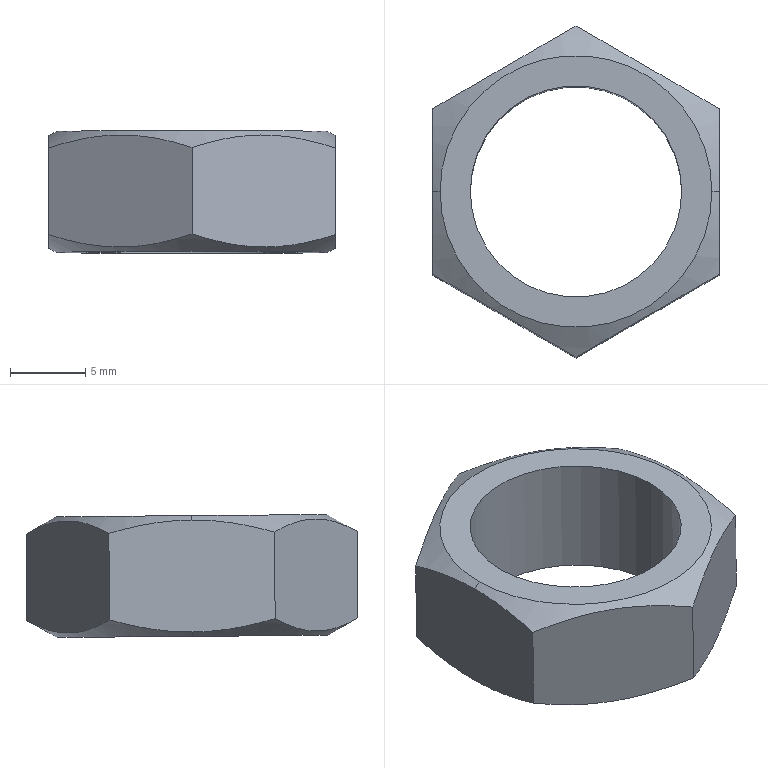Component | SolidWorks | CG1UN40-50Nut-1 | 1 solid | 14 faces | box 19 x 21.98 x 8.14 mm | volume 1229 mm3 | plane 8 | cone 4 | cylinder 2 | commonest cylinder face diameters 14 x2
STEP:
#1=CARTESIAN_POINT('',(7.598,4.142,0.1182));
#2=VERTEX_POINT('',#1);
#3=CARTESIAN_POINT('',(8.15,4.142,0.1182));
#4=VERTEX_POINT('',#3);
#5=CARTESIAN_POINT('',(7.874,4.142,0.1182));
#6=DIRECTION('',(-0.,0.008055,1.));
#7=DIRECTION('',(-1.,0.,-0.));
#8=AXIS2_PLACEMENT_3D('',#5,#6,#7);
#9=CIRCLE('',#8,0.2756);
#10=EDGE_CURVE('',#2,#4,#9,.T.);
#11=ORIENTED_EDGE('',*,*,#10,.F.);
#12=CARTESIAN_POINT('',(7.598,4.145,0.4332));
#13=VERTEX_POINT('',#12);
#14=CARTESIAN_POINT('',(7.598,4.144,0.2757));
#15=DIRECTION('',(-0.,0.008055,1.));
#16=VECTOR('',#15,39.37);
#17=LINE('',#14,#16);
#18=EDGE_CURVE('',#2,#13,#17,.T.);
#19=ORIENTED_EDGE('',*,*,#18,.T.);
#20=CARTESIAN_POINT('',(8.15,4.145,0.4332));
#21=VERTEX_POINT('',#20);
#22=CARTESIAN_POINT('',(7.874,4.145,0.4332));
#23=DIRECTION('',(0.,-0.008055,-1.));
#24=DIRECTION('',(1.,-0.,0.));
#25=AXIS2_PLACEMENT_3D('',#22,#23,#24);
#26=CIRCLE('',#25,0.2756);
#27=EDGE_CURVE('',#21,#13,#26,.T.);
#28=ORIENTED_EDGE('',*,*,#27,.F.);
#29=CARTESIAN_POINT('',(8.15,4.144,0.2757));
#30=DIRECTION('',(-0.,0.008055,1.));
#31=VECTOR('',#30,39.37);
#32=LINE('',#29,#31);
#33=EDGE_CURVE('',#4,#21,#32,.T.);
#34=ORIENTED_EDGE('',*,*,#33,.F.);
#35=EDGE_LOOP('',(#11,#19,#28,#34));
#36=FACE_OUTER_BOUND('',#35,.T.);
#37=CARTESIAN_POINT('',(7.874,4.144,0.2757));
#38=DIRECTION('',(-0.,0.008055,1.));
#39=DIRECTION('',(1.,0.,0.));
#40=AXIS2_PLACEMENT_3D('',#37,#38,#39);
#41=CYLINDRICAL_SURFACE('',#40,0.2756);
#42=ADVANCED_FACE('',(#36),#41,.F.);
#43=CARTESIAN_POINT('',(8.228,4.142,0.1182));
#44=VERTEX_POINT('',#43);
#45=CARTESIAN_POINT('',(7.52,4.142,0.1182));
#46=VERTEX_POINT('',#45);
#47=CARTESIAN_POINT('',(7.874,4.142,0.1182));
#48=DIRECTION('',(-0.,0.008055,1.));
#49=DIRECTION('',(1.,0.,0.));
#50=AXIS2_PLACEMENT_3D('',#47,#48,#49);
#51=CIRCLE('',#50,0.3543);
#52=EDGE_CURVE('',#44,#46,#51,.T.);
#53=ORIENTED_EDGE('',*,*,#52,.T.);
#54=CARTESIAN_POINT('',(7.5,4.142,0.1296));
#55=VERTEX_POINT('',#54);
#56=CARTESIAN_POINT('',(7.442,4.143,0.1633));
#57=DIRECTION('',(-0.866,0.004027,0.5));
#58=VECTOR('',#57,39.37);
#59=LINE('',#56,#58);
#60=EDGE_CURVE('',#46,#55,#59,.T.);
#61=ORIENTED_EDGE('',*,*,#60,.T.);
#62=CARTESIAN_POINT('',(7.5,4.359,0.1613));
#63=VERTEX_POINT('',#62);
#64=CARTESIAN_POINT('',(7.5,4.142,0.1296));
#65=CARTESIAN_POINT('',(7.5,4.161,0.1295));
#66=CARTESIAN_POINT('',(7.5,4.179,0.1301));
#67=CARTESIAN_POINT('',(7.5,4.216,0.1329));
#68=CARTESIAN_POINT('',(7.5,4.234,0.135));
#69=CARTESIAN_POINT('',(7.5,4.288,0.1433));
#70=CARTESIAN_POINT('',(7.5,4.323,0.1514));
#71=CARTESIAN_POINT('',(7.5,4.359,0.1613));
#72=B_SPLINE_CURVE_WITH_KNOTS('',3,(#64,#65,#66,#67,#68,#69,#70,#71),.UNSPECIFIED.,.F.,.F.,(4,2,2,4),(0.00555,0.006932,0.008314,0.01108),.UNSPECIFIED.);
#73=EDGE_CURVE('',#55,#63,#72,.T.);
#74=ORIENTED_EDGE('',*,*,#73,.T.);
#75=CARTESIAN_POINT('',(7.874,4.575,0.1595));
#76=VERTEX_POINT('',#75);
#77=CARTESIAN_POINT('',(7.5,4.359,0.1613));
#78=CARTESIAN_POINT('',(7.531,4.376,0.1509));
#79=CARTESIAN_POINT('',(7.561,4.394,0.1424));
#80=CARTESIAN_POINT('',(7.623,4.43,0.1305));
#81=CARTESIAN_POINT('',(7.655,4.448,0.1272));
#82=CARTESIAN_POINT('',(7.703,4.475,0.1269));
#83=CARTESIAN_POINT('',(7.719,4.484,0.1276));
#84=CARTESIAN_POINT('',(7.75,4.503,0.1305));
#85=CARTESIAN_POINT('',(7.766,4.512,0.1327));
#86=CARTESIAN_POINT('',(7.813,4.539,0.1412));
#87=CARTESIAN_POINT('',(7.843,4.557,0.1495));
#88=CARTESIAN_POINT('',(7.874,4.575,0.1595));
#89=B_SPLINE_CURVE_WITH_KNOTS('',3,(#77,#78,#79,#80,#81,#82,#83,#84,#85,#86,#87,#88),.UNSPECIFIED.,.F.,.F.,(4,2,2,2,2,4),(0.,0.00277,0.005539,0.006924,0.008309,0.01108),.UNSPECIFIED.);
#90=EDGE_CURVE('',#63,#76,#89,.T.);
#91=ORIENTED_EDGE('',*,*,#90,.T.);
#92=CARTESIAN_POINT('',(8.248,4.359,0.1613));
#93=VERTEX_POINT('',#92);
#94=CARTESIAN_POINT('',(7.874,4.575,0.1595));
#95=CARTESIAN_POINT('',(7.905,4.557,0.1495));
#96=CARTESIAN_POINT('',(7.935,4.539,0.1412));
#97=CARTESIAN_POINT('',(7.997,4.503,0.1299));
#98=CARTESIAN_POINT('',(8.029,4.485,0.1269));
#99=CARTESIAN_POINT('',(8.077,4.457,0.1271));
#100=CARTESIAN_POINT('',(8.093,4.448,0.1279));
#101=CARTESIAN_POINT('',(8.124,4.43,0.1311));
#102=CARTESIAN_POINT('',(8.14,4.421,0.1334));
#103=CARTESIAN_POINT('',(8.187,4.394,0.1424));
#104=CARTESIAN_POINT('',(8.217,4.376,0.1509));
#105=CARTESIAN_POINT('',(8.248,4.359,0.1613));
#106=B_SPLINE_CURVE_WITH_KNOTS('',3,(#94,#95,#96,#97,#98,#99,#100,#101,#102,#103,#104,#105),.UNSPECIFIED.,.F.,.F.,(4,2,2,2,2,4),(0.,0.00277,0.005539,0.006924,0.008309,0.01108),.UNSPECIFIED.);
#107=EDGE_CURVE('',#76,#93,#106,.T.);
#108=ORIENTED_EDGE('',*,*,#107,.T.);
#109=CARTESIAN_POINT('',(8.248,4.142,0.1296));
#110=VERTEX_POINT('',#109);
#111=CARTESIAN_POINT('',(8.248,4.359,0.1613));
#112=CARTESIAN_POINT('',(8.248,4.323,0.1514));
#113=CARTESIAN_POINT('',(8.248,4.288,0.1432));
#114=CARTESIAN_POINT('',(8.248,4.216,0.1322));
#115=CARTESIAN_POINT('',(8.248,4.179,0.1293));
#116=CARTESIAN_POINT('',(8.248,4.142,0.1296));
#117=B_SPLINE_CURVE_WITH_KNOTS('',3,(#111,#112,#113,#114,#115,#116),.UNSPECIFIED.,.F.,.F.,(4,2,4),(0.,0.002775,0.00555),.UNSPECIFIED.);
#118=EDGE_CURVE('',#93,#110,#117,.T.);
#119=ORIENTED_EDGE('',*,*,#118,.T.);
#120=CARTESIAN_POINT('',(8.306,4.143,0.1633));
#121=DIRECTION('',(0.866,0.004027,0.5));
#122=VECTOR('',#121,39.37);
#123=LINE('',#120,#122);
#124=EDGE_CURVE('',#44,#110,#123,.T.);
#125=ORIENTED_EDGE('',*,*,#124,.F.);
#126=EDGE_LOOP('',(#53,#61,#74,#91,#108,#119,#125));
#127=FACE_OUTER_BOUND('',#126,.T.);
#128=CARTESIAN_POINT('',(7.874,4.143,0.1633));
#129=DIRECTION('',(-0.,0.008055,1.));
#130=DIRECTION('',(1.,0.,0.));
#131=AXIS2_PLACEMENT_3D('',#128,#129,#130);
#132=CONICAL_SURFACE('',#131,0.4323,1.047);
#133=ADVANCED_FACE('',(#127),#132,.T.);
#134=CARTESIAN_POINT('',(8.228,4.145,0.4332));
#135=VERTEX_POINT('',#134);
#136=CARTESIAN_POINT('',(7.52,4.145,0.4332));
#137=VERTEX_POINT('',#136);
#138=CARTESIAN_POINT('',(7.874,4.145,0.4332));
#139=DIRECTION('',(-0.,0.008055,1.));
#140=DIRECTION('',(-1.,0.,-0.));
#141=AXIS2_PLACEMENT_3D('',#138,#139,#140);
#142=CIRCLE('',#141,0.3543);
#143=EDGE_CURVE('',#135,#137,#142,.T.);
#144=ORIENTED_EDGE('',*,*,#143,.F.);
#145=CARTESIAN_POINT('',(8.248,4.145,0.4218));
#146=VERTEX_POINT('',#145);
#147=CARTESIAN_POINT('',(8.306,4.144,0.3881));
#148=DIRECTION('',(0.866,-0.004027,-0.5));
#149=VECTOR('',#148,39.37);
#150=LINE('',#147,#149);
#151=EDGE_CURVE('',#135,#146,#150,.T.);
#152=ORIENTED_EDGE('',*,*,#151,.T.);
#153=CARTESIAN_POINT('',(8.248,4.36,0.3867));
#154=VERTEX_POINT('',#153);
#155=CARTESIAN_POINT('',(8.248,4.145,0.4218));
#156=CARTESIAN_POINT('',(8.248,4.163,0.4217));
#157=CARTESIAN_POINT('',(8.248,4.181,0.4207));
#158=CARTESIAN_POINT('',(8.248,4.218,0.4174));
#159=CARTESIAN_POINT('',(8.248,4.236,0.415));
#160=CARTESIAN_POINT('',(8.248,4.29,0.4058));
#161=CARTESIAN_POINT('',(8.248,4.325,0.3971));
#162=CARTESIAN_POINT('',(8.248,4.36,0.3867));
#163=B_SPLINE_CURVE_WITH_KNOTS('',3,(#155,#156,#157,#158,#159,#160,#161,#162),.UNSPECIFIED.,.F.,.F.,(4,2,2,4),(0.00555,0.006932,0.008314,0.01108),.UNSPECIFIED.);
#164=EDGE_CURVE('',#146,#154,#163,.T.);
#165=ORIENTED_EDGE('',*,*,#164,.T.);
#166=CARTESIAN_POINT('',(7.874,4.576,0.3849));
#167=VERTEX_POINT('',#166);
#168=CARTESIAN_POINT('',(8.248,4.36,0.3867));
#169=CARTESIAN_POINT('',(8.217,4.378,0.3967));
#170=CARTESIAN_POINT('',(8.187,4.396,0.405));
#171=CARTESIAN_POINT('',(8.125,4.432,0.4163));
#172=CARTESIAN_POINT('',(8.093,4.45,0.4193));
#173=CARTESIAN_POINT('',(8.045,4.478,0.4192));
#174=CARTESIAN_POINT('',(8.03,4.487,0.4183));
#175=CARTESIAN_POINT('',(7.998,4.505,0.4151));
#176=CARTESIAN_POINT('',(7.982,4.514,0.4128));
#177=CARTESIAN_POINT('',(7.935,4.541,0.4038));
#178=CARTESIAN_POINT('',(7.905,4.559,0.3953));
#179=CARTESIAN_POINT('',(7.874,4.576,0.3849));
#180=B_SPLINE_CURVE_WITH_KNOTS('',3,(#168,#169,#170,#171,#172,#173,#174,#175,#176,#177,#178,#179),.UNSPECIFIED.,.F.,.F.,(4,2,2,2,2,4),(0.,0.00277,0.005539,0.006924,0.008309,0.01108),.UNSPECIFIED.);
#181=EDGE_CURVE('',#154,#167,#180,.T.);
#182=ORIENTED_EDGE('',*,*,#181,.T.);
#183=CARTESIAN_POINT('',(7.5,4.36,0.3867));
#184=VERTEX_POINT('',#183);
#185=CARTESIAN_POINT('',(7.874,4.576,0.3849));
#186=CARTESIAN_POINT('',(7.843,4.559,0.3953));
#187=CARTESIAN_POINT('',(7.813,4.541,0.4038));
#188=CARTESIAN_POINT('',(7.751,4.505,0.4157));
#189=CARTESIAN_POINT('',(7.719,4.487,0.419));
#190=CARTESIAN_POINT('',(7.671,4.46,0.4193));
#191=CARTESIAN_POINT('',(7.655,4.45,0.4186));
#192=CARTESIAN_POINT('',(7.624,4.432,0.4157));
#193=CARTESIAN_POINT('',(7.608,4.423,0.4135));
#194=CARTESIAN_POINT('',(7.561,4.396,0.405));
#195=CARTESIAN_POINT('',(7.531,4.378,0.3967));
#196=CARTESIAN_POINT('',(7.5,4.36,0.3867));
#197=B_SPLINE_CURVE_WITH_KNOTS('',3,(#185,#186,#187,#188,#189,#190,#191,#192,#193,#194,#195,#196),.UNSPECIFIED.,.F.,.F.,(4,2,2,2,2,4),(0.,0.00277,0.005539,0.006924,0.008309,0.01108),.UNSPECIFIED.);
#198=EDGE_CURVE('',#167,#184,#197,.T.);
#199=ORIENTED_EDGE('',*,*,#198,.T.);
#200=CARTESIAN_POINT('',(7.5,4.145,0.4218));
#201=VERTEX_POINT('',#200);
#202=CARTESIAN_POINT('',(7.5,4.36,0.3867));
#203=CARTESIAN_POINT('',(7.5,4.325,0.3972));
#204=CARTESIAN_POINT('',(7.5,4.29,0.4058));
#205=CARTESIAN_POINT('',(7.5,4.218,0.418));
#206=CARTESIAN_POINT('',(7.5,4.182,0.4215));
#207=CARTESIAN_POINT('',(7.5,4.145,0.4218));
#208=B_SPLINE_CURVE_WITH_KNOTS('',3,(#202,#203,#204,#205,#206,#207),.UNSPECIFIED.,.F.,.F.,(4,2,4),(0.,0.002775,0.00555),.UNSPECIFIED.);
#209=EDGE_CURVE('',#184,#201,#208,.T.);
#210=ORIENTED_EDGE('',*,*,#209,.T.);
#211=CARTESIAN_POINT('',(7.442,4.144,0.3881));
#212=DIRECTION('',(-0.866,-0.004027,-0.5));
#213=VECTOR('',#212,39.37);
#214=LINE('',#211,#213);
#215=EDGE_CURVE('',#137,#201,#214,.T.);
#216=ORIENTED_EDGE('',*,*,#215,.F.);
#217=EDGE_LOOP('',(#144,#152,#165,#182,#199,#210,#216));
#218=FACE_OUTER_BOUND('',#217,.T.);
#219=CARTESIAN_POINT('',(7.874,4.144,0.3881));
#220=DIRECTION('',(0.,-0.008055,-1.));
#221=DIRECTION('',(-1.,0.,-0.));
#222=AXIS2_PLACEMENT_3D('',#219,#220,#221);
#223=CONICAL_SURFACE('',#222,0.4323,1.047);
#224=ADVANCED_FACE('',(#218),#223,.T.);
#225=ORIENTED_EDGE('',*,*,#18,.F.);
#226=CARTESIAN_POINT('',(7.874,4.142,0.1182));
#227=DIRECTION('',(-0.,0.008055,1.));
#228=DIRECTION('',(-1.,0.,-0.));
#229=AXIS2_PLACEMENT_3D('',#226,#227,#228);
#230=CIRCLE('',#229,0.2756);
#231=EDGE_CURVE('',#4,#2,#230,.T.);
#232=ORIENTED_EDGE('',*,*,#231,.F.);
#233=ORIENTED_EDGE('',*,*,#33,.T.);
#234=CARTESIAN_POINT('',(7.874,4.145,0.4332));
#235=DIRECTION('',(0.,-0.008055,-1.));
#236=DIRECTION('',(1.,0.,0.));
#237=AXIS2_PLACEMENT_3D('',#234,#235,#236);
#238=CIRCLE('',#237,0.2756);
#239=EDGE_CURVE('',#13,#21,#238,.T.);
#240=ORIENTED_EDGE('',*,*,#239,.F.);
#241=EDGE_LOOP('',(#225,#232,#233,#240));
#242=FACE_OUTER_BOUND('',#241,.T.);
#243=CARTESIAN_POINT('',(7.874,4.144,0.2757));
#244=DIRECTION('',(-0.,0.008055,1.));
#245=DIRECTION('',(1.,0.,0.));
#246=AXIS2_PLACEMENT_3D('',#243,#244,#245);
#247=CYLINDRICAL_SURFACE('',#246,0.2756);
#248=ADVANCED_FACE('',(#242),#247,.F.);
#249=ORIENTED_EDGE('',*,*,#231,.T.);
#250=ORIENTED_EDGE('',*,*,#10,.T.);
#251=EDGE_LOOP('',(#249,#250));
#252=FACE_BOUND('',#251,.T.);
#253=ORIENTED_EDGE('',*,*,#52,.F.);
#254=CARTESIAN_POINT('',(7.874,4.142,0.1182));
#255=DIRECTION('',(-0.,0.008055,1.));
#256=DIRECTION('',(1.,0.,0.));
#257=AXIS2_PLACEMENT_3D('',#254,#255,#256);
#258=CIRCLE('',#257,0.3543);
#259=EDGE_CURVE('',#46,#44,#258,.T.);
#260=ORIENTED_EDGE('',*,*,#259,.F.);
#261=EDGE_LOOP('',(#253,#260));
#262=FACE_OUTER_BOUND('',#261,.T.);
#263=CARTESIAN_POINT('',(7.874,4.142,0.1182));
#264=DIRECTION('',(-0.,0.008055,1.));
#265=DIRECTION('',(1.,0.,0.));
#266=AXIS2_PLACEMENT_3D('',#263,#264,#265);
#267=PLANE('',#266);
#268=ADVANCED_FACE('',(#252,#262),#267,.F.);
#269=ORIENTED_EDGE('',*,*,#27,.T.);
#270=ORIENTED_EDGE('',*,*,#239,.T.);
#271=EDGE_LOOP('',(#269,#270));
#272=FACE_BOUND('',#271,.T.);
#273=CARTESIAN_POINT('',(7.874,4.145,0.4332));
#274=DIRECTION('',(-0.,0.008055,1.));
#275=DIRECTION('',(-1.,-0.,-0.));
#276=AXIS2_PLACEMENT_3D('',#273,#274,#275);
#277=CIRCLE('',#276,0.3543);
#278=EDGE_CURVE('',#137,#135,#277,.T.);
#279=ORIENTED_EDGE('',*,*,#278,.T.);
#280=ORIENTED_EDGE('',*,*,#143,.T.);
#281=EDGE_LOOP('',(#279,#280));
#282=FACE_OUTER_BOUND('',#281,.T.);
#283=CARTESIAN_POINT('',(7.874,4.145,0.4332));
#284=DIRECTION('',(-0.,0.008055,1.));
#285=DIRECTION('',(1.,0.,0.));
#286=AXIS2_PLACEMENT_3D('',#283,#284,#285);
#287=PLANE('',#286);
#288=ADVANCED_FACE('',(#272,#282),#287,.T.);
#289=ORIENTED_EDGE('',*,*,#60,.F.);
#290=ORIENTED_EDGE('',*,*,#259,.T.);
#291=ORIENTED_EDGE('',*,*,#124,.T.);
#292=CARTESIAN_POINT('',(8.248,3.927,0.1647));
#293=VERTEX_POINT('',#292);
#294=CARTESIAN_POINT('',(8.248,4.142,0.1296));
#295=CARTESIAN_POINT('',(8.248,4.124,0.1297));
#296=CARTESIAN_POINT('',(8.248,4.106,0.1307));
#297=CARTESIAN_POINT('',(8.248,4.069,0.134));
#298=CARTESIAN_POINT('',(8.248,4.051,0.1364));
#299=CARTESIAN_POINT('',(8.248,3.997,0.1456));
#300=CARTESIAN_POINT('',(8.248,3.962,0.1543));
#301=CARTESIAN_POINT('',(8.248,3.927,0.1647));
#302=B_SPLINE_CURVE_WITH_KNOTS('',3,(#294,#295,#296,#297,#298,#299,#300,#301),.UNSPECIFIED.,.F.,.F.,(4,2,2,4),(0.00555,0.006932,0.008314,0.01108),.UNSPECIFIED.);
#303=EDGE_CURVE('',#110,#293,#302,.T.);
#304=ORIENTED_EDGE('',*,*,#303,.T.);
#305=CARTESIAN_POINT('',(7.874,3.711,0.1665));
#306=VERTEX_POINT('',#305);
#307=CARTESIAN_POINT('',(8.248,3.927,0.1647));
#308=CARTESIAN_POINT('',(8.217,3.909,0.1547));
#309=CARTESIAN_POINT('',(8.187,3.891,0.1465));
#310=CARTESIAN_POINT('',(8.125,3.855,0.1351));
#311=CARTESIAN_POINT('',(8.093,3.837,0.1321));
#312=CARTESIAN_POINT('',(8.045,3.81,0.1323));
#313=CARTESIAN_POINT('',(8.03,3.8,0.1331));
#314=CARTESIAN_POINT('',(7.998,3.782,0.1363));
#315=CARTESIAN_POINT('',(7.982,3.773,0.1386));
#316=CARTESIAN_POINT('',(7.935,3.746,0.1476));
#317=CARTESIAN_POINT('',(7.905,3.728,0.1562));
#318=CARTESIAN_POINT('',(7.874,3.711,0.1665));
#319=B_SPLINE_CURVE_WITH_KNOTS('',3,(#307,#308,#309,#310,#311,#312,#313,#314,#315,#316,#317,#318),.UNSPECIFIED.,.F.,.F.,(4,2,2,2,2,4),(0.,0.00277,0.005539,0.006924,0.008309,0.01108),.UNSPECIFIED.);
#320=EDGE_CURVE('',#293,#306,#319,.T.);
#321=ORIENTED_EDGE('',*,*,#320,.T.);
#322=CARTESIAN_POINT('',(7.5,3.927,0.1647));
#323=VERTEX_POINT('',#322);
#324=CARTESIAN_POINT('',(7.874,3.711,0.1665));
#325=CARTESIAN_POINT('',(7.843,3.728,0.1562));
#326=CARTESIAN_POINT('',(7.813,3.746,0.1476));
#327=CARTESIAN_POINT('',(7.751,3.782,0.1357));
#328=CARTESIAN_POINT('',(7.719,3.8,0.1324));
#329=CARTESIAN_POINT('',(7.671,3.827,0.1321));
#330=CARTESIAN_POINT('',(7.655,3.837,0.1328));
#331=CARTESIAN_POINT('',(7.624,3.855,0.1357));
#332=CARTESIAN_POINT('',(7.608,3.864,0.1379));
#333=CARTESIAN_POINT('',(7.561,3.891,0.1464));
#334=CARTESIAN_POINT('',(7.531,3.909,0.1547));
#335=CARTESIAN_POINT('',(7.5,3.927,0.1647));
#336=B_SPLINE_CURVE_WITH_KNOTS('',3,(#324,#325,#326,#327,#328,#329,#330,#331,#332,#333,#334,#335),.UNSPECIFIED.,.F.,.F.,(4,2,2,2,2,4),(0.,0.00277,0.005539,0.006924,0.008309,0.01108),.UNSPECIFIED.);
#337=EDGE_CURVE('',#306,#323,#336,.T.);
#338=ORIENTED_EDGE('',*,*,#337,.T.);
#339=CARTESIAN_POINT('',(7.5,3.927,0.1647));
#340=CARTESIAN_POINT('',(7.5,3.962,0.1543));
#341=CARTESIAN_POINT('',(7.5,3.997,0.1456));
#342=CARTESIAN_POINT('',(7.5,4.069,0.1334));
#343=CARTESIAN_POINT('',(7.5,4.106,0.1299));
#344=CARTESIAN_POINT('',(7.5,4.142,0.1296));
#345=B_SPLINE_CURVE_WITH_KNOTS('',3,(#339,#340,#341,#342,#343,#344),.UNSPECIFIED.,.F.,.F.,(4,2,4),(0.,0.002775,0.00555),.UNSPECIFIED.);
#346=EDGE_CURVE('',#323,#55,#345,.T.);
#347=ORIENTED_EDGE('',*,*,#346,.T.);
#348=EDGE_LOOP('',(#289,#290,#291,#304,#321,#338,#347));
#349=FACE_OUTER_BOUND('',#348,.T.);
#350=CARTESIAN_POINT('',(7.874,4.143,0.1633));
#351=DIRECTION('',(-0.,0.008055,1.));
#352=DIRECTION('',(1.,0.,0.));
#353=AXIS2_PLACEMENT_3D('',#350,#351,#352);
#354=CONICAL_SURFACE('',#353,0.4323,1.047);
#355=ADVANCED_FACE('',(#349),#354,.T.);
#356=ORIENTED_EDGE('',*,*,#151,.F.);
#357=ORIENTED_EDGE('',*,*,#278,.F.);
#358=ORIENTED_EDGE('',*,*,#215,.T.);
#359=CARTESIAN_POINT('',(7.5,3.929,0.3902));
#360=VERTEX_POINT('',#359);
#361=CARTESIAN_POINT('',(7.5,4.145,0.4218));
#362=CARTESIAN_POINT('',(7.5,4.126,0.422));
#363=CARTESIAN_POINT('',(7.5,4.108,0.4213));
#364=CARTESIAN_POINT('',(7.5,4.072,0.4186));
#365=CARTESIAN_POINT('',(7.5,4.053,0.4164));
#366=CARTESIAN_POINT('',(7.5,3.999,0.4082));
#367=CARTESIAN_POINT('',(7.5,3.964,0.4));
#368=CARTESIAN_POINT('',(7.5,3.929,0.3902));
#369=B_SPLINE_CURVE_WITH_KNOTS('',3,(#361,#362,#363,#364,#365,#366,#367,#368),.UNSPECIFIED.,.F.,.F.,(4,2,2,4),(0.00555,0.006932,0.008314,0.01108),.UNSPECIFIED.);
#370=EDGE_CURVE('',#201,#360,#369,.T.);
#371=ORIENTED_EDGE('',*,*,#370,.T.);
#372=CARTESIAN_POINT('',(7.874,3.713,0.3919));
#373=VERTEX_POINT('',#372);
#374=CARTESIAN_POINT('',(7.5,3.929,0.3902));
#375=CARTESIAN_POINT('',(7.531,3.911,0.4005));
#376=CARTESIAN_POINT('',(7.561,3.893,0.409));
#377=CARTESIAN_POINT('',(7.623,3.858,0.4209));
#378=CARTESIAN_POINT('',(7.655,3.839,0.4243));
#379=CARTESIAN_POINT('',(7.703,3.812,0.4245));
#380=CARTESIAN_POINT('',(7.719,3.803,0.4238));
#381=CARTESIAN_POINT('',(7.75,3.784,0.4209));
#382=CARTESIAN_POINT('',(7.766,3.775,0.4187));
#383=CARTESIAN_POINT('',(7.813,3.748,0.4102));
#384=CARTESIAN_POINT('',(7.843,3.73,0.4019));
#385=CARTESIAN_POINT('',(7.874,3.713,0.3919));
#386=B_SPLINE_CURVE_WITH_KNOTS('',3,(#374,#375,#376,#377,#378,#379,#380,#381,#382,#383,#384,#385),.UNSPECIFIED.,.F.,.F.,(4,2,2,2,2,4),(0.,0.00277,0.005539,0.006924,0.008309,0.01108),.UNSPECIFIED.);
#387=EDGE_CURVE('',#360,#373,#386,.T.);
#388=ORIENTED_EDGE('',*,*,#387,.T.);
#389=CARTESIAN_POINT('',(8.248,3.929,0.3902));
#390=VERTEX_POINT('',#389);
#391=CARTESIAN_POINT('',(7.874,3.713,0.3919));
#392=CARTESIAN_POINT('',(7.905,3.73,0.4019));
#393=CARTESIAN_POINT('',(7.935,3.748,0.4102));
#394=CARTESIAN_POINT('',(7.997,3.784,0.4215));
#395=CARTESIAN_POINT('',(8.029,3.802,0.4246));
#396=CARTESIAN_POINT('',(8.077,3.83,0.4244));
#397=CARTESIAN_POINT('',(8.093,3.839,0.4235));
#398=CARTESIAN_POINT('',(8.124,3.857,0.4203));
#399=CARTESIAN_POINT('',(8.14,3.866,0.418));
#400=CARTESIAN_POINT('',(8.187,3.893,0.409));
#401=CARTESIAN_POINT('',(8.217,3.911,0.4005));
#402=CARTESIAN_POINT('',(8.248,3.929,0.3902));
#403=B_SPLINE_CURVE_WITH_KNOTS('',3,(#391,#392,#393,#394,#395,#396,#397,#398,#399,#400,#401,#402),.UNSPECIFIED.,.F.,.F.,(4,2,2,2,2,4),(0.,0.00277,0.005539,0.006924,0.008309,0.01108),.UNSPECIFIED.);
#404=EDGE_CURVE('',#373,#390,#403,.T.);
#405=ORIENTED_EDGE('',*,*,#404,.T.);
#406=CARTESIAN_POINT('',(8.248,3.929,0.3902));
#407=CARTESIAN_POINT('',(8.248,3.964,0.4001));
#408=CARTESIAN_POINT('',(8.248,4.,0.4082));
#409=CARTESIAN_POINT('',(8.248,4.072,0.4192));
#410=CARTESIAN_POINT('',(8.248,4.108,0.4221));
#411=CARTESIAN_POINT('',(8.248,4.145,0.4218));
#412=B_SPLINE_CURVE_WITH_KNOTS('',3,(#406,#407,#408,#409,#410,#411),.UNSPECIFIED.,.F.,.F.,(4,2,4),(0.,0.002775,0.00555),.UNSPECIFIED.);
#413=EDGE_CURVE('',#390,#146,#412,.T.);
#414=ORIENTED_EDGE('',*,*,#413,.T.);
#415=EDGE_LOOP('',(#356,#357,#358,#371,#388,#405,#414));
#416=FACE_OUTER_BOUND('',#415,.T.);
#417=CARTESIAN_POINT('',(7.874,4.144,0.3881));
#418=DIRECTION('',(0.,-0.008055,-1.));
#419=DIRECTION('',(-1.,0.,-0.));
#420=AXIS2_PLACEMENT_3D('',#417,#418,#419);
#421=CONICAL_SURFACE('',#420,0.4323,1.047);
#422=ADVANCED_FACE('',(#416),#421,.T.);
#423=ORIENTED_EDGE('',*,*,#404,.F.);
#424=CARTESIAN_POINT('',(7.874,3.713,0.4367));
#425=DIRECTION('',(0.,-0.008055,-1.));
#426=VECTOR('',#425,39.37);
#427=LINE('',#424,#426);
#428=EDGE_CURVE('',#373,#306,#427,.T.);
#429=ORIENTED_EDGE('',*,*,#428,.T.);
#430=ORIENTED_EDGE('',*,*,#320,.F.);
#431=CARTESIAN_POINT('',(8.248,3.929,0.4349));
#432=DIRECTION('',(-0.,0.008055,1.));
#433=VECTOR('',#432,39.37);
#434=LINE('',#431,#433);
#435=EDGE_CURVE('',#293,#390,#434,.T.);
#436=ORIENTED_EDGE('',*,*,#435,.T.);
#437=EDGE_LOOP('',(#423,#429,#430,#436));
#438=FACE_OUTER_BOUND('',#437,.T.);
#439=CARTESIAN_POINT('',(7.874,3.713,0.4367));
#440=DIRECTION('',(0.5,-0.866,0.006976));
#441=DIRECTION('',(0.866,0.5,-0.004027));
#442=AXIS2_PLACEMENT_3D('',#439,#440,#441);
#443=PLANE('',#442);
#444=ADVANCED_FACE('',(#438),#443,.T.);
#445=ORIENTED_EDGE('',*,*,#413,.F.);
#446=ORIENTED_EDGE('',*,*,#435,.F.);
#447=ORIENTED_EDGE('',*,*,#303,.F.);
#448=ORIENTED_EDGE('',*,*,#118,.F.);
#449=CARTESIAN_POINT('',(8.248,4.361,0.4314));
#450=DIRECTION('',(-0.,0.008055,1.));
#451=VECTOR('',#450,39.37);
#452=LINE('',#449,#451);
#453=EDGE_CURVE('',#93,#154,#452,.T.);
#454=ORIENTED_EDGE('',*,*,#453,.T.);
#455=ORIENTED_EDGE('',*,*,#164,.F.);
#456=EDGE_LOOP('',(#445,#446,#447,#448,#454,#455));
#457=FACE_OUTER_BOUND('',#456,.T.);
#458=CARTESIAN_POINT('',(8.248,3.929,0.4349));
#459=DIRECTION('',(1.,0.,0.));
#460=DIRECTION('',(0.,-0.008055,-1.));
#461=AXIS2_PLACEMENT_3D('',#458,#459,#460);
#462=PLANE('',#461);
#463=ADVANCED_FACE('',(#457),#462,.T.);
#464=ORIENTED_EDGE('',*,*,#181,.F.);
#465=ORIENTED_EDGE('',*,*,#453,.F.);
#466=ORIENTED_EDGE('',*,*,#107,.F.);
#467=CARTESIAN_POINT('',(7.874,4.577,0.4297));
#468=DIRECTION('',(-0.,0.008055,1.));
#469=VECTOR('',#468,39.37);
#470=LINE('',#467,#469);
#471=EDGE_CURVE('',#76,#167,#470,.T.);
#472=ORIENTED_EDGE('',*,*,#471,.T.);
#473=EDGE_LOOP('',(#464,#465,#466,#472));
#474=FACE_OUTER_BOUND('',#473,.T.);
#475=CARTESIAN_POINT('',(8.248,4.361,0.4314));
#476=DIRECTION('',(0.5,0.866,-0.006976));
#477=DIRECTION('',(-0.866,0.5,-0.004027));
#478=AXIS2_PLACEMENT_3D('',#475,#476,#477);
#479=PLANE('',#478);
#480=ADVANCED_FACE('',(#474),#479,.T.);
#481=ORIENTED_EDGE('',*,*,#198,.F.);
#482=ORIENTED_EDGE('',*,*,#471,.F.);
#483=ORIENTED_EDGE('',*,*,#90,.F.);
#484=CARTESIAN_POINT('',(7.5,4.361,0.4314));
#485=DIRECTION('',(-0.,0.008055,1.));
#486=VECTOR('',#485,39.37);
#487=LINE('',#484,#486);
#488=EDGE_CURVE('',#63,#184,#487,.T.);
#489=ORIENTED_EDGE('',*,*,#488,.T.);
#490=EDGE_LOOP('',(#481,#482,#483,#489));
#491=FACE_OUTER_BOUND('',#490,.T.);
#492=CARTESIAN_POINT('',(7.874,4.577,0.4297));
#493=DIRECTION('',(-0.5,0.866,-0.006976));
#494=DIRECTION('',(-0.866,-0.5,0.004027));
#495=AXIS2_PLACEMENT_3D('',#492,#493,#494);
#496=PLANE('',#495);
#497=ADVANCED_FACE('',(#491),#496,.T.);
#498=ORIENTED_EDGE('',*,*,#209,.F.);
#499=ORIENTED_EDGE('',*,*,#488,.F.);
#500=ORIENTED_EDGE('',*,*,#73,.F.);
#501=ORIENTED_EDGE('',*,*,#346,.F.);
#502=CARTESIAN_POINT('',(7.5,3.929,0.4349));
#503=DIRECTION('',(-0.,0.008055,1.));
#504=VECTOR('',#503,39.37);
#505=LINE('',#502,#504);
#506=EDGE_CURVE('',#323,#360,#505,.T.);
#507=ORIENTED_EDGE('',*,*,#506,.T.);
#508=ORIENTED_EDGE('',*,*,#370,.F.);
#509=EDGE_LOOP('',(#498,#499,#500,#501,#507,#508));
#510=FACE_OUTER_BOUND('',#509,.T.);
#511=CARTESIAN_POINT('',(7.5,4.361,0.4314));
#512=DIRECTION('',(-1.,-0.,-0.));
#513=DIRECTION('',(-0.,0.008055,1.));
#514=AXIS2_PLACEMENT_3D('',#511,#512,#513);
#515=PLANE('',#514);
#516=ADVANCED_FACE('',(#510),#515,.T.);
#517=ORIENTED_EDGE('',*,*,#387,.F.);
#518=ORIENTED_EDGE('',*,*,#506,.F.);
#519=ORIENTED_EDGE('',*,*,#337,.F.);
#520=ORIENTED_EDGE('',*,*,#428,.F.);
#521=EDGE_LOOP('',(#517,#518,#519,#520));
#522=FACE_OUTER_BOUND('',#521,.T.);
#523=CARTESIAN_POINT('',(7.5,3.929,0.4349));
#524=DIRECTION('',(-0.5,-0.866,0.006976));
#525=DIRECTION('',(0.866,-0.5,0.004027));
#526=AXIS2_PLACEMENT_3D('',#523,#524,#525);
#527=PLANE('',#526);
#528=ADVANCED_FACE('',(#522),#527,.T.);
#529=CLOSED_SHELL('',(#42,#133,#224,#248,#268,#288,#355,#422,#444,#463,#480,#497,#516,#528));
#530=MANIFOLD_SOLID_BREP('',#529);
#531=CARTESIAN_POINT('',(0.,0.,0.));
#532=DIRECTION('',(0.,0.,1.));
#533=DIRECTION('',(1.,0.,0.));
#534=AXIS2_PLACEMENT_3D('',#531,#532,#533);
#535=(LENGTH_UNIT()NAMED_UNIT(*)SI_UNIT($,.METRE.));
#536=LENGTH_MEASURE_WITH_UNIT(LENGTH_MEASURE(0.0254),#535);
#537=DIMENSIONAL_EXPONENTS(1.,0.,0.,0.,0.,0.,0.);
#538=(CONVERSION_BASED_UNIT('',#536)LENGTH_UNIT()NAMED_UNIT(#537));
#539=UNCERTAINTY_MEASURE_WITH_UNIT(LENGTH_MEASURE(0.00001),#538,'','');
#540=(NAMED_UNIT(*)PLANE_ANGLE_UNIT()SI_UNIT($,.RADIAN.));
#541=(NAMED_UNIT(*)SI_UNIT($,.STERADIAN.)SOLID_ANGLE_UNIT());
#542=(GEOMETRIC_REPRESENTATION_CONTEXT(3)GLOBAL_UNCERTAINTY_ASSIGNED_CONTEXT((#539))GLOBAL_UNIT_ASSIGNED_CONTEXT((#538,#540,#541))REPRESENTATION_CONTEXT('',''));
#543=ADVANCED_BREP_SHAPE_REPRESENTATION('',(#530,#534),#542);
#544=COLOUR_RGB('',0.7922,0.8196,0.9333);
#545=FILL_AREA_STYLE_COLOUR('',#544);
#546=FILL_AREA_STYLE('',(#545));
#547=SURFACE_STYLE_FILL_AREA(#546);
#548=SURFACE_SIDE_STYLE('',(#547));
#549=SURFACE_STYLE_USAGE(.BOTH.,#548);
#550=PRESENTATION_STYLE_ASSIGNMENT((#549));
#551=STYLED_ITEM('',(#550),#530);
#552=PRESENTATION_LAYER_ASSIGNMENT('','',(#551));
#553=(LENGTH_UNIT()NAMED_UNIT(*)SI_UNIT($,.METRE.));
#554=LENGTH_MEASURE_WITH_UNIT(LENGTH_MEASURE(0.0254),#553);
#555=DIMENSIONAL_EXPONENTS(1.,0.,0.,0.,0.,0.,0.);
#556=(CONVERSION_BASED_UNIT('',#554)LENGTH_UNIT()NAMED_UNIT(#555));
#557=UNCERTAINTY_MEASURE_WITH_UNIT(LENGTH_MEASURE(0.00001),#556,'','');
#558=(NAMED_UNIT(*)PLANE_ANGLE_UNIT()SI_UNIT($,.RADIAN.));
#559=(NAMED_UNIT(*)SI_UNIT($,.STERADIAN.)SOLID_ANGLE_UNIT());
#560=(GEOMETRIC_REPRESENTATION_CONTEXT(3)GLOBAL_UNCERTAINTY_ASSIGNED_CONTEXT((#557))GLOBAL_UNIT_ASSIGNED_CONTEXT((#556,#558,#559))REPRESENTATION_CONTEXT('',''));
#561=MECHANICAL_DESIGN_GEOMETRIC_PRESENTATION_REPRESENTATION('',(#551),#560);